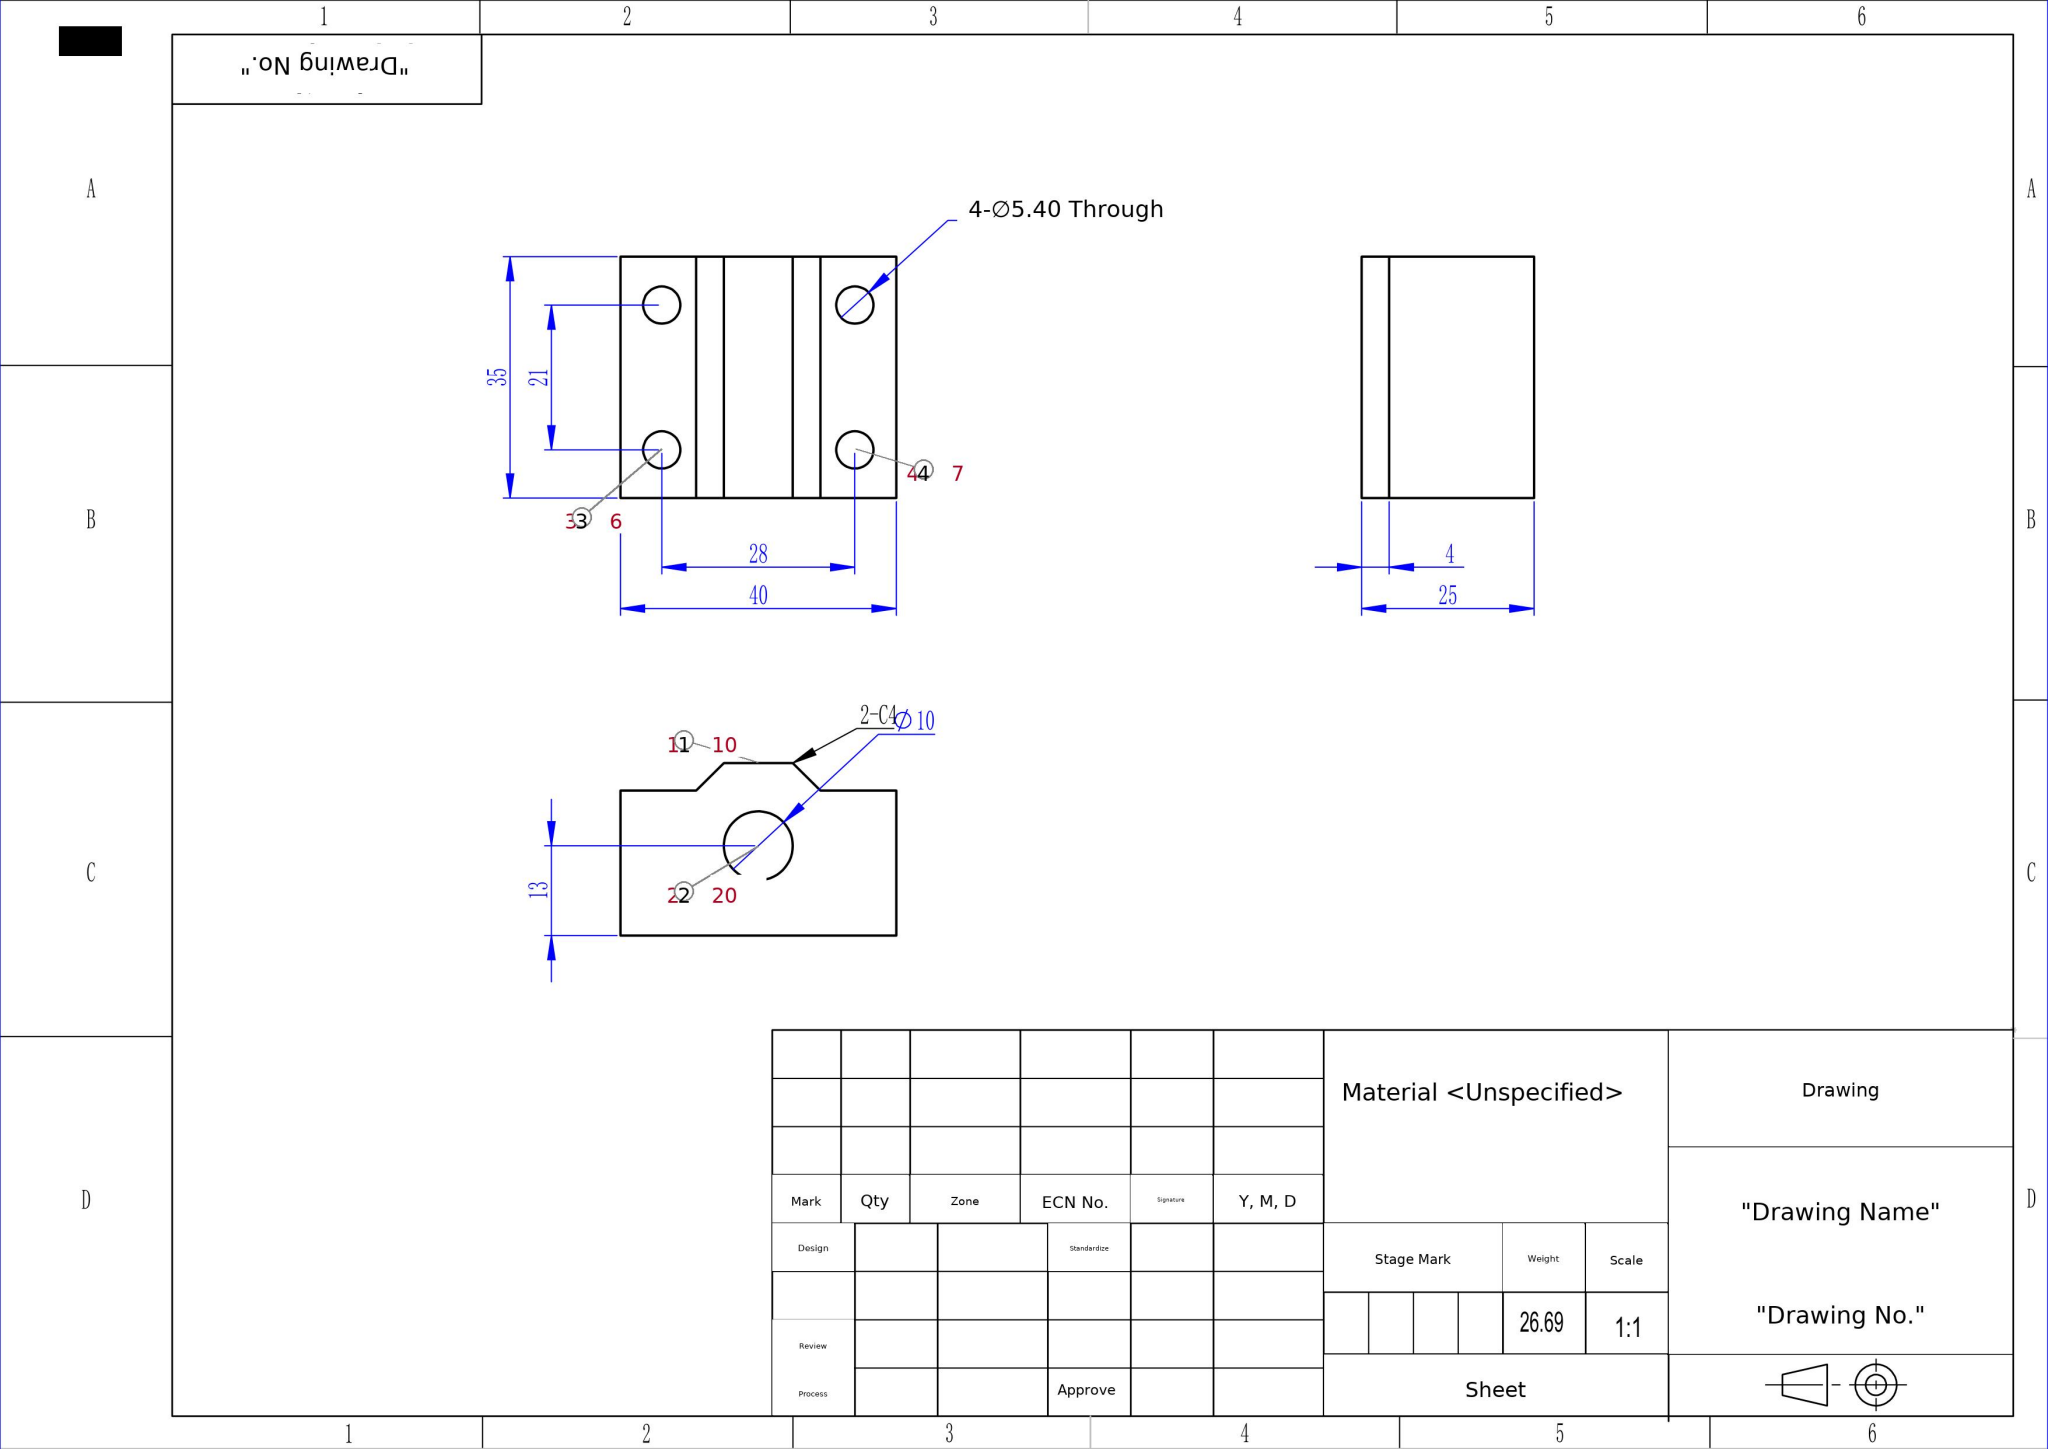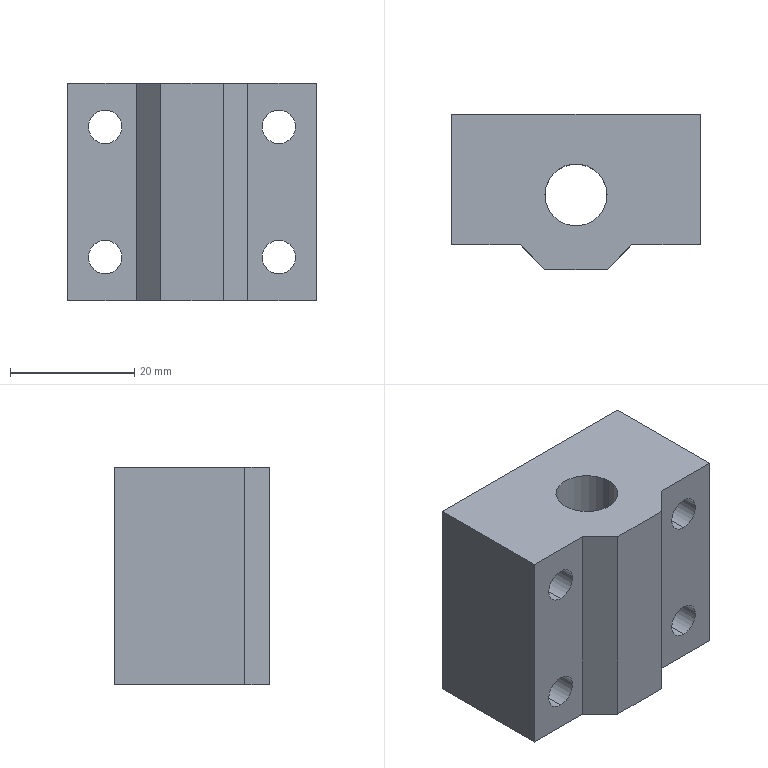Part | SolidWorks | mm | 1 solid | 20 faces | box 40 x 25 x 35 mm | volume 26687 mm3 | cylinder 10 | plane 10 | commonest cylinder face diameters 5.4 x8 10 x2
STEP:
#1=CARTESIAN_POINT('',(-14.,-8.,4.3));
#2=VERTEX_POINT('',#1);
#3=CARTESIAN_POINT('',(-14.,-8.,9.7));
#4=VERTEX_POINT('',#3);
#5=CARTESIAN_POINT('',(-14.,-8.,7.));
#6=DIRECTION('',(0.,1.,0.));
#7=DIRECTION('',(0.,0.,1.));
#8=AXIS2_PLACEMENT_3D('',#5,#6,#7);
#9=CIRCLE('',#8,2.7);
#10=EDGE_CURVE('',#2,#4,#9,.T.);
#11=ORIENTED_EDGE('',*,*,#10,.F.);
#12=CARTESIAN_POINT('',(-14.,13.,4.3));
#13=VERTEX_POINT('',#12);
#14=CARTESIAN_POINT('',(-14.,-12.,4.3));
#15=DIRECTION('',(0.,1.,0.));
#16=VECTOR('',#15,1000.);
#17=LINE('',#14,#16);
#18=EDGE_CURVE('',#2,#13,#17,.T.);
#19=ORIENTED_EDGE('',*,*,#18,.T.);
#20=CARTESIAN_POINT('',(-14.,13.,9.7));
#21=VERTEX_POINT('',#20);
#22=CARTESIAN_POINT('',(-14.,13.,7.));
#23=DIRECTION('',(0.,1.,0.));
#24=DIRECTION('',(0.,0.,1.));
#25=AXIS2_PLACEMENT_3D('',#22,#23,#24);
#26=CIRCLE('',#25,2.7);
#27=EDGE_CURVE('',#13,#21,#26,.T.);
#28=ORIENTED_EDGE('',*,*,#27,.T.);
#29=CARTESIAN_POINT('',(-14.,-12.,9.7));
#30=DIRECTION('',(0.,1.,0.));
#31=VECTOR('',#30,1000.);
#32=LINE('',#29,#31);
#33=EDGE_CURVE('',#4,#21,#32,.T.);
#34=ORIENTED_EDGE('',*,*,#33,.F.);
#35=EDGE_LOOP('',(#11,#19,#28,#34));
#36=FACE_OUTER_BOUND('',#35,.T.);
#37=CARTESIAN_POINT('',(-14.,-12.,7.));
#38=DIRECTION('',(0.,1.,0.));
#39=DIRECTION('',(0.,0.,1.));
#40=AXIS2_PLACEMENT_3D('',#37,#38,#39);
#41=CYLINDRICAL_SURFACE('',#40,2.7);
#42=ADVANCED_FACE('',(#36),#41,.F.);
#43=CARTESIAN_POINT('',(14.,-8.,4.3));
#44=VERTEX_POINT('',#43);
#45=CARTESIAN_POINT('',(14.,-8.,9.7));
#46=VERTEX_POINT('',#45);
#47=CARTESIAN_POINT('',(14.,-8.,7.));
#48=DIRECTION('',(0.,1.,0.));
#49=DIRECTION('',(0.,0.,1.));
#50=AXIS2_PLACEMENT_3D('',#47,#48,#49);
#51=CIRCLE('',#50,2.7);
#52=EDGE_CURVE('',#44,#46,#51,.T.);
#53=ORIENTED_EDGE('',*,*,#52,.F.);
#54=CARTESIAN_POINT('',(14.,13.,4.3));
#55=VERTEX_POINT('',#54);
#56=CARTESIAN_POINT('',(14.,-12.,4.3));
#57=DIRECTION('',(0.,1.,0.));
#58=VECTOR('',#57,1000.);
#59=LINE('',#56,#58);
#60=EDGE_CURVE('',#44,#55,#59,.T.);
#61=ORIENTED_EDGE('',*,*,#60,.T.);
#62=CARTESIAN_POINT('',(14.,13.,9.7));
#63=VERTEX_POINT('',#62);
#64=CARTESIAN_POINT('',(14.,13.,7.));
#65=DIRECTION('',(0.,1.,0.));
#66=DIRECTION('',(0.,0.,1.));
#67=AXIS2_PLACEMENT_3D('',#64,#65,#66);
#68=CIRCLE('',#67,2.7);
#69=EDGE_CURVE('',#55,#63,#68,.T.);
#70=ORIENTED_EDGE('',*,*,#69,.T.);
#71=CARTESIAN_POINT('',(14.,-12.,9.7));
#72=DIRECTION('',(0.,1.,0.));
#73=VECTOR('',#72,1000.);
#74=LINE('',#71,#73);
#75=EDGE_CURVE('',#46,#63,#74,.T.);
#76=ORIENTED_EDGE('',*,*,#75,.F.);
#77=EDGE_LOOP('',(#53,#61,#70,#76));
#78=FACE_OUTER_BOUND('',#77,.T.);
#79=CARTESIAN_POINT('',(14.,-12.,7.));
#80=DIRECTION('',(0.,1.,0.));
#81=DIRECTION('',(0.,0.,1.));
#82=AXIS2_PLACEMENT_3D('',#79,#80,#81);
#83=CYLINDRICAL_SURFACE('',#82,2.7);
#84=ADVANCED_FACE('',(#78),#83,.F.);
#85=CARTESIAN_POINT('',(14.,-8.,25.3));
#86=VERTEX_POINT('',#85);
#87=CARTESIAN_POINT('',(14.,-8.,30.7));
#88=VERTEX_POINT('',#87);
#89=CARTESIAN_POINT('',(14.,-8.,28.));
#90=DIRECTION('',(0.,1.,0.));
#91=DIRECTION('',(0.,0.,1.));
#92=AXIS2_PLACEMENT_3D('',#89,#90,#91);
#93=CIRCLE('',#92,2.7);
#94=EDGE_CURVE('',#86,#88,#93,.T.);
#95=ORIENTED_EDGE('',*,*,#94,.F.);
#96=CARTESIAN_POINT('',(14.,13.,25.3));
#97=VERTEX_POINT('',#96);
#98=CARTESIAN_POINT('',(14.,-12.,25.3));
#99=DIRECTION('',(0.,1.,0.));
#100=VECTOR('',#99,1000.);
#101=LINE('',#98,#100);
#102=EDGE_CURVE('',#86,#97,#101,.T.);
#103=ORIENTED_EDGE('',*,*,#102,.T.);
#104=CARTESIAN_POINT('',(14.,13.,30.7));
#105=VERTEX_POINT('',#104);
#106=CARTESIAN_POINT('',(14.,13.,28.));
#107=DIRECTION('',(0.,1.,0.));
#108=DIRECTION('',(0.,0.,1.));
#109=AXIS2_PLACEMENT_3D('',#106,#107,#108);
#110=CIRCLE('',#109,2.7);
#111=EDGE_CURVE('',#97,#105,#110,.T.);
#112=ORIENTED_EDGE('',*,*,#111,.T.);
#113=CARTESIAN_POINT('',(14.,-12.,30.7));
#114=DIRECTION('',(0.,1.,0.));
#115=VECTOR('',#114,1000.);
#116=LINE('',#113,#115);
#117=EDGE_CURVE('',#88,#105,#116,.T.);
#118=ORIENTED_EDGE('',*,*,#117,.F.);
#119=EDGE_LOOP('',(#95,#103,#112,#118));
#120=FACE_OUTER_BOUND('',#119,.T.);
#121=CARTESIAN_POINT('',(14.,-12.,28.));
#122=DIRECTION('',(0.,1.,0.));
#123=DIRECTION('',(0.,0.,1.));
#124=AXIS2_PLACEMENT_3D('',#121,#122,#123);
#125=CYLINDRICAL_SURFACE('',#124,2.7);
#126=ADVANCED_FACE('',(#120),#125,.F.);
#127=CARTESIAN_POINT('',(-14.,-8.,25.3));
#128=VERTEX_POINT('',#127);
#129=CARTESIAN_POINT('',(-14.,-8.,30.7));
#130=VERTEX_POINT('',#129);
#131=CARTESIAN_POINT('',(-14.,-8.,28.));
#132=DIRECTION('',(0.,1.,0.));
#133=DIRECTION('',(0.,0.,1.));
#134=AXIS2_PLACEMENT_3D('',#131,#132,#133);
#135=CIRCLE('',#134,2.7);
#136=EDGE_CURVE('',#128,#130,#135,.T.);
#137=ORIENTED_EDGE('',*,*,#136,.F.);
#138=CARTESIAN_POINT('',(-14.,13.,25.3));
#139=VERTEX_POINT('',#138);
#140=CARTESIAN_POINT('',(-14.,-12.,25.3));
#141=DIRECTION('',(0.,1.,0.));
#142=VECTOR('',#141,1000.);
#143=LINE('',#140,#142);
#144=EDGE_CURVE('',#128,#139,#143,.T.);
#145=ORIENTED_EDGE('',*,*,#144,.T.);
#146=CARTESIAN_POINT('',(-14.,13.,30.7));
#147=VERTEX_POINT('',#146);
#148=CARTESIAN_POINT('',(-14.,13.,28.));
#149=DIRECTION('',(0.,1.,0.));
#150=DIRECTION('',(0.,0.,1.));
#151=AXIS2_PLACEMENT_3D('',#148,#149,#150);
#152=CIRCLE('',#151,2.7);
#153=EDGE_CURVE('',#139,#147,#152,.T.);
#154=ORIENTED_EDGE('',*,*,#153,.T.);
#155=CARTESIAN_POINT('',(-14.,-12.,30.7));
#156=DIRECTION('',(0.,1.,0.));
#157=VECTOR('',#156,1000.);
#158=LINE('',#155,#157);
#159=EDGE_CURVE('',#130,#147,#158,.T.);
#160=ORIENTED_EDGE('',*,*,#159,.F.);
#161=EDGE_LOOP('',(#137,#145,#154,#160));
#162=FACE_OUTER_BOUND('',#161,.T.);
#163=CARTESIAN_POINT('',(-14.,-12.,28.));
#164=DIRECTION('',(0.,1.,0.));
#165=DIRECTION('',(0.,0.,1.));
#166=AXIS2_PLACEMENT_3D('',#163,#164,#165);
#167=CYLINDRICAL_SURFACE('',#166,2.7);
#168=ADVANCED_FACE('',(#162),#167,.F.);
#169=CARTESIAN_POINT('',(-5.,0.,35.));
#170=VERTEX_POINT('',#169);
#171=CARTESIAN_POINT('',(5.,0.,35.));
#172=VERTEX_POINT('',#171);
#173=CARTESIAN_POINT('',(0.,0.,35.));
#174=DIRECTION('',(0.,0.,1.));
#175=DIRECTION('',(1.,0.,0.));
#176=AXIS2_PLACEMENT_3D('',#173,#174,#175);
#177=CIRCLE('',#176,5.);
#178=EDGE_CURVE('',#170,#172,#177,.T.);
#179=ORIENTED_EDGE('',*,*,#178,.T.);
#180=CARTESIAN_POINT('',(5.,0.,0.));
#181=VERTEX_POINT('',#180);
#182=CARTESIAN_POINT('',(5.,0.,35.));
#183=DIRECTION('',(0.,0.,-1.));
#184=VECTOR('',#183,1000.);
#185=LINE('',#182,#184);
#186=EDGE_CURVE('',#172,#181,#185,.T.);
#187=ORIENTED_EDGE('',*,*,#186,.T.);
#188=CARTESIAN_POINT('',(-5.,0.,0.));
#189=VERTEX_POINT('',#188);
#190=CARTESIAN_POINT('',(0.,0.,0.));
#191=DIRECTION('',(0.,0.,1.));
#192=DIRECTION('',(1.,0.,0.));
#193=AXIS2_PLACEMENT_3D('',#190,#191,#192);
#194=CIRCLE('',#193,5.);
#195=EDGE_CURVE('',#189,#181,#194,.T.);
#196=ORIENTED_EDGE('',*,*,#195,.F.);
#197=CARTESIAN_POINT('',(-5.,0.,35.));
#198=DIRECTION('',(0.,0.,-1.));
#199=VECTOR('',#198,1000.);
#200=LINE('',#197,#199);
#201=EDGE_CURVE('',#170,#189,#200,.T.);
#202=ORIENTED_EDGE('',*,*,#201,.F.);
#203=EDGE_LOOP('',(#179,#187,#196,#202));
#204=FACE_OUTER_BOUND('',#203,.T.);
#205=CARTESIAN_POINT('',(0.,0.,35.));
#206=DIRECTION('',(0.,0.,-1.));
#207=DIRECTION('',(-1.,0.,0.));
#208=AXIS2_PLACEMENT_3D('',#205,#206,#207);
#209=CYLINDRICAL_SURFACE('',#208,5.);
#210=ADVANCED_FACE('',(#204),#209,.F.);
#211=CARTESIAN_POINT('',(-20.,13.,35.));
#212=VERTEX_POINT('',#211);
#213=CARTESIAN_POINT('',(-20.,-8.,35.));
#214=VERTEX_POINT('',#213);
#215=CARTESIAN_POINT('',(-20.,13.,35.));
#216=DIRECTION('',(0.,-1.,0.));
#217=VECTOR('',#216,1000.);
#218=LINE('',#215,#217);
#219=EDGE_CURVE('',#212,#214,#218,.T.);
#220=ORIENTED_EDGE('',*,*,#219,.T.);
#221=CARTESIAN_POINT('',(-9.,-8.,35.));
#222=VERTEX_POINT('',#221);
#223=CARTESIAN_POINT('',(-20.,-8.,35.));
#224=DIRECTION('',(1.,0.,0.));
#225=VECTOR('',#224,1000.);
#226=LINE('',#223,#225);
#227=EDGE_CURVE('',#214,#222,#226,.T.);
#228=ORIENTED_EDGE('',*,*,#227,.T.);
#229=CARTESIAN_POINT('',(-5.,-12.,35.));
#230=VERTEX_POINT('',#229);
#231=CARTESIAN_POINT('',(-5.,-12.,35.));
#232=DIRECTION('',(0.7071,-0.7071,0.));
#233=VECTOR('',#232,1000.);
#234=LINE('',#231,#233);
#235=EDGE_CURVE('',#222,#230,#234,.T.);
#236=ORIENTED_EDGE('',*,*,#235,.T.);
#237=CARTESIAN_POINT('',(5.,-12.,35.));
#238=VERTEX_POINT('',#237);
#239=CARTESIAN_POINT('',(-5.,-12.,35.));
#240=DIRECTION('',(1.,0.,0.));
#241=VECTOR('',#240,1000.);
#242=LINE('',#239,#241);
#243=EDGE_CURVE('',#230,#238,#242,.T.);
#244=ORIENTED_EDGE('',*,*,#243,.T.);
#245=CARTESIAN_POINT('',(9.,-8.,35.));
#246=VERTEX_POINT('',#245);
#247=CARTESIAN_POINT('',(9.,-8.,35.));
#248=DIRECTION('',(0.7071,0.7071,0.));
#249=VECTOR('',#248,1000.);
#250=LINE('',#247,#249);
#251=EDGE_CURVE('',#238,#246,#250,.T.);
#252=ORIENTED_EDGE('',*,*,#251,.T.);
#253=CARTESIAN_POINT('',(20.,-8.,35.));
#254=VERTEX_POINT('',#253);
#255=CARTESIAN_POINT('',(5.,-8.,35.));
#256=DIRECTION('',(1.,0.,0.));
#257=VECTOR('',#256,1000.);
#258=LINE('',#255,#257);
#259=EDGE_CURVE('',#246,#254,#258,.T.);
#260=ORIENTED_EDGE('',*,*,#259,.T.);
#261=CARTESIAN_POINT('',(20.,13.,35.));
#262=VERTEX_POINT('',#261);
#263=CARTESIAN_POINT('',(20.,13.,35.));
#264=DIRECTION('',(0.,1.,0.));
#265=VECTOR('',#264,1000.);
#266=LINE('',#263,#265);
#267=EDGE_CURVE('',#254,#262,#266,.T.);
#268=ORIENTED_EDGE('',*,*,#267,.T.);
#269=CARTESIAN_POINT('',(-20.,13.,35.));
#270=DIRECTION('',(-1.,0.,0.));
#271=VECTOR('',#270,1000.);
#272=LINE('',#269,#271);
#273=EDGE_CURVE('',#262,#212,#272,.T.);
#274=ORIENTED_EDGE('',*,*,#273,.T.);
#275=EDGE_LOOP('',(#220,#228,#236,#244,#252,#260,#268,#274));
#276=FACE_OUTER_BOUND('',#275,.T.);
#277=ORIENTED_EDGE('',*,*,#178,.F.);
#278=CARTESIAN_POINT('',(0.,0.,35.));
#279=DIRECTION('',(0.,0.,1.));
#280=DIRECTION('',(1.,0.,0.));
#281=AXIS2_PLACEMENT_3D('',#278,#279,#280);
#282=CIRCLE('',#281,5.);
#283=EDGE_CURVE('',#172,#170,#282,.T.);
#284=ORIENTED_EDGE('',*,*,#283,.F.);
#285=EDGE_LOOP('',(#277,#284));
#286=FACE_BOUND('',#285,.T.);
#287=CARTESIAN_POINT('',(0.,0.,35.));
#288=DIRECTION('',(0.,0.,1.));
#289=DIRECTION('',(1.,0.,0.));
#290=AXIS2_PLACEMENT_3D('',#287,#288,#289);
#291=PLANE('',#290);
#292=ADVANCED_FACE('',(#276,#286),#291,.T.);
#293=CARTESIAN_POINT('',(-20.,13.,0.));
#294=VERTEX_POINT('',#293);
#295=CARTESIAN_POINT('',(-20.,-8.,0.));
#296=VERTEX_POINT('',#295);
#297=CARTESIAN_POINT('',(-20.,13.,0.));
#298=DIRECTION('',(0.,-1.,0.));
#299=VECTOR('',#298,1000.);
#300=LINE('',#297,#299);
#301=EDGE_CURVE('',#294,#296,#300,.T.);
#302=ORIENTED_EDGE('',*,*,#301,.F.);
#303=CARTESIAN_POINT('',(20.,13.,0.));
#304=VERTEX_POINT('',#303);
#305=CARTESIAN_POINT('',(-20.,13.,0.));
#306=DIRECTION('',(-1.,0.,0.));
#307=VECTOR('',#306,1000.);
#308=LINE('',#305,#307);
#309=EDGE_CURVE('',#304,#294,#308,.T.);
#310=ORIENTED_EDGE('',*,*,#309,.F.);
#311=CARTESIAN_POINT('',(20.,-8.,0.));
#312=VERTEX_POINT('',#311);
#313=CARTESIAN_POINT('',(20.,13.,0.));
#314=DIRECTION('',(0.,1.,0.));
#315=VECTOR('',#314,1000.);
#316=LINE('',#313,#315);
#317=EDGE_CURVE('',#312,#304,#316,.T.);
#318=ORIENTED_EDGE('',*,*,#317,.F.);
#319=CARTESIAN_POINT('',(9.,-8.,0.));
#320=VERTEX_POINT('',#319);
#321=CARTESIAN_POINT('',(5.,-8.,0.));
#322=DIRECTION('',(1.,0.,0.));
#323=VECTOR('',#322,1000.);
#324=LINE('',#321,#323);
#325=EDGE_CURVE('',#320,#312,#324,.T.);
#326=ORIENTED_EDGE('',*,*,#325,.F.);
#327=CARTESIAN_POINT('',(5.,-12.,0.));
#328=VERTEX_POINT('',#327);
#329=CARTESIAN_POINT('',(8.5,-8.5,0.));
#330=DIRECTION('',(-0.7071,-0.7071,0.));
#331=VECTOR('',#330,1000.);
#332=LINE('',#329,#331);
#333=EDGE_CURVE('',#320,#328,#332,.T.);
#334=ORIENTED_EDGE('',*,*,#333,.T.);
#335=CARTESIAN_POINT('',(-5.,-12.,0.));
#336=VERTEX_POINT('',#335);
#337=CARTESIAN_POINT('',(-5.,-12.,0.));
#338=DIRECTION('',(1.,0.,0.));
#339=VECTOR('',#338,1000.);
#340=LINE('',#337,#339);
#341=EDGE_CURVE('',#336,#328,#340,.T.);
#342=ORIENTED_EDGE('',*,*,#341,.F.);
#343=CARTESIAN_POINT('',(-9.,-8.,0.));
#344=VERTEX_POINT('',#343);
#345=CARTESIAN_POINT('',(-8.5,-8.5,0.));
#346=DIRECTION('',(-0.7071,0.7071,0.));
#347=VECTOR('',#346,1000.);
#348=LINE('',#345,#347);
#349=EDGE_CURVE('',#336,#344,#348,.T.);
#350=ORIENTED_EDGE('',*,*,#349,.T.);
#351=CARTESIAN_POINT('',(-20.,-8.,0.));
#352=DIRECTION('',(1.,0.,0.));
#353=VECTOR('',#352,1000.);
#354=LINE('',#351,#353);
#355=EDGE_CURVE('',#296,#344,#354,.T.);
#356=ORIENTED_EDGE('',*,*,#355,.F.);
#357=EDGE_LOOP('',(#302,#310,#318,#326,#334,#342,#350,#356));
#358=FACE_OUTER_BOUND('',#357,.T.);
#359=ORIENTED_EDGE('',*,*,#195,.T.);
#360=CARTESIAN_POINT('',(0.,0.,0.));
#361=DIRECTION('',(0.,0.,1.));
#362=DIRECTION('',(1.,0.,0.));
#363=AXIS2_PLACEMENT_3D('',#360,#361,#362);
#364=CIRCLE('',#363,5.);
#365=EDGE_CURVE('',#181,#189,#364,.T.);
#366=ORIENTED_EDGE('',*,*,#365,.T.);
#367=EDGE_LOOP('',(#359,#366));
#368=FACE_BOUND('',#367,.T.);
#369=CARTESIAN_POINT('',(0.,0.,0.));
#370=DIRECTION('',(0.,0.,1.));
#371=DIRECTION('',(1.,0.,0.));
#372=AXIS2_PLACEMENT_3D('',#369,#370,#371);
#373=PLANE('',#372);
#374=ADVANCED_FACE('',(#358,#368),#373,.F.);
#375=ORIENTED_EDGE('',*,*,#301,.T.);
#376=CARTESIAN_POINT('',(-20.,-8.,35.));
#377=DIRECTION('',(0.,0.,-1.));
#378=VECTOR('',#377,1000.);
#379=LINE('',#376,#378);
#380=EDGE_CURVE('',#214,#296,#379,.T.);
#381=ORIENTED_EDGE('',*,*,#380,.F.);
#382=ORIENTED_EDGE('',*,*,#219,.F.);
#383=CARTESIAN_POINT('',(-20.,13.,35.));
#384=DIRECTION('',(0.,0.,-1.));
#385=VECTOR('',#384,1000.);
#386=LINE('',#383,#385);
#387=EDGE_CURVE('',#212,#294,#386,.T.);
#388=ORIENTED_EDGE('',*,*,#387,.T.);
#389=EDGE_LOOP('',(#375,#381,#382,#388));
#390=FACE_OUTER_BOUND('',#389,.T.);
#391=CARTESIAN_POINT('',(-20.,13.,35.));
#392=DIRECTION('',(1.,0.,0.));
#393=DIRECTION('',(-0.,1.,0.));
#394=AXIS2_PLACEMENT_3D('',#391,#392,#393);
#395=PLANE('',#394);
#396=ADVANCED_FACE('',(#390),#395,.F.);
#397=CARTESIAN_POINT('',(-14.,-8.,7.));
#398=DIRECTION('',(0.,1.,0.));
#399=DIRECTION('',(0.,0.,1.));
#400=AXIS2_PLACEMENT_3D('',#397,#398,#399);
#401=CIRCLE('',#400,2.7);
#402=EDGE_CURVE('',#4,#2,#401,.T.);
#403=ORIENTED_EDGE('',*,*,#402,.T.);
#404=ORIENTED_EDGE('',*,*,#10,.T.);
#405=EDGE_LOOP('',(#403,#404));
#406=FACE_BOUND('',#405,.T.);
#407=CARTESIAN_POINT('',(-14.,-8.,28.));
#408=DIRECTION('',(0.,1.,0.));
#409=DIRECTION('',(0.,0.,1.));
#410=AXIS2_PLACEMENT_3D('',#407,#408,#409);
#411=CIRCLE('',#410,2.7);
#412=EDGE_CURVE('',#130,#128,#411,.T.);
#413=ORIENTED_EDGE('',*,*,#412,.T.);
#414=ORIENTED_EDGE('',*,*,#136,.T.);
#415=EDGE_LOOP('',(#413,#414));
#416=FACE_BOUND('',#415,.T.);
#417=ORIENTED_EDGE('',*,*,#355,.T.);
#418=CARTESIAN_POINT('',(-9.,-8.,35.));
#419=DIRECTION('',(0.,0.,1.));
#420=VECTOR('',#419,1000.);
#421=LINE('',#418,#420);
#422=EDGE_CURVE('',#344,#222,#421,.T.);
#423=ORIENTED_EDGE('',*,*,#422,.T.);
#424=ORIENTED_EDGE('',*,*,#227,.F.);
#425=ORIENTED_EDGE('',*,*,#380,.T.);
#426=EDGE_LOOP('',(#417,#423,#424,#425));
#427=FACE_OUTER_BOUND('',#426,.T.);
#428=CARTESIAN_POINT('',(-20.,-8.,35.));
#429=DIRECTION('',(0.,1.,0.));
#430=DIRECTION('',(0.,0.,1.));
#431=AXIS2_PLACEMENT_3D('',#428,#429,#430);
#432=PLANE('',#431);
#433=ADVANCED_FACE('',(#406,#416,#427),#432,.F.);
#434=ORIENTED_EDGE('',*,*,#341,.T.);
#435=CARTESIAN_POINT('',(5.,-12.,35.));
#436=DIRECTION('',(0.,0.,-1.));
#437=VECTOR('',#436,1000.);
#438=LINE('',#435,#437);
#439=EDGE_CURVE('',#238,#328,#438,.T.);
#440=ORIENTED_EDGE('',*,*,#439,.F.);
#441=ORIENTED_EDGE('',*,*,#243,.F.);
#442=CARTESIAN_POINT('',(-5.,-12.,35.));
#443=DIRECTION('',(0.,0.,-1.));
#444=VECTOR('',#443,1000.);
#445=LINE('',#442,#444);
#446=EDGE_CURVE('',#230,#336,#445,.T.);
#447=ORIENTED_EDGE('',*,*,#446,.T.);
#448=EDGE_LOOP('',(#434,#440,#441,#447));
#449=FACE_OUTER_BOUND('',#448,.T.);
#450=CARTESIAN_POINT('',(-5.,-12.,35.));
#451=DIRECTION('',(0.,1.,0.));
#452=DIRECTION('',(0.,0.,1.));
#453=AXIS2_PLACEMENT_3D('',#450,#451,#452);
#454=PLANE('',#453);
#455=ADVANCED_FACE('',(#449),#454,.F.);
#456=CARTESIAN_POINT('',(14.,-8.,7.));
#457=DIRECTION('',(0.,1.,0.));
#458=DIRECTION('',(0.,0.,1.));
#459=AXIS2_PLACEMENT_3D('',#456,#457,#458);
#460=CIRCLE('',#459,2.7);
#461=EDGE_CURVE('',#46,#44,#460,.T.);
#462=ORIENTED_EDGE('',*,*,#461,.T.);
#463=ORIENTED_EDGE('',*,*,#52,.T.);
#464=EDGE_LOOP('',(#462,#463));
#465=FACE_BOUND('',#464,.T.);
#466=CARTESIAN_POINT('',(14.,-8.,28.));
#467=DIRECTION('',(0.,1.,0.));
#468=DIRECTION('',(0.,0.,1.));
#469=AXIS2_PLACEMENT_3D('',#466,#467,#468);
#470=CIRCLE('',#469,2.7);
#471=EDGE_CURVE('',#88,#86,#470,.T.);
#472=ORIENTED_EDGE('',*,*,#471,.T.);
#473=ORIENTED_EDGE('',*,*,#94,.T.);
#474=EDGE_LOOP('',(#472,#473));
#475=FACE_BOUND('',#474,.T.);
#476=ORIENTED_EDGE('',*,*,#259,.F.);
#477=CARTESIAN_POINT('',(9.,-8.,0.));
#478=DIRECTION('',(0.,0.,-1.));
#479=VECTOR('',#478,1000.);
#480=LINE('',#477,#479);
#481=EDGE_CURVE('',#246,#320,#480,.T.);
#482=ORIENTED_EDGE('',*,*,#481,.T.);
#483=ORIENTED_EDGE('',*,*,#325,.T.);
#484=CARTESIAN_POINT('',(20.,-8.,35.));
#485=DIRECTION('',(0.,0.,-1.));
#486=VECTOR('',#485,1000.);
#487=LINE('',#484,#486);
#488=EDGE_CURVE('',#254,#312,#487,.T.);
#489=ORIENTED_EDGE('',*,*,#488,.F.);
#490=EDGE_LOOP('',(#476,#482,#483,#489));
#491=FACE_OUTER_BOUND('',#490,.T.);
#492=CARTESIAN_POINT('',(5.,-8.,35.));
#493=DIRECTION('',(0.,1.,0.));
#494=DIRECTION('',(0.,0.,1.));
#495=AXIS2_PLACEMENT_3D('',#492,#493,#494);
#496=PLANE('',#495);
#497=ADVANCED_FACE('',(#465,#475,#491),#496,.F.);
#498=ORIENTED_EDGE('',*,*,#317,.T.);
#499=CARTESIAN_POINT('',(20.,13.,35.));
#500=DIRECTION('',(0.,0.,-1.));
#501=VECTOR('',#500,1000.);
#502=LINE('',#499,#501);
#503=EDGE_CURVE('',#262,#304,#502,.T.);
#504=ORIENTED_EDGE('',*,*,#503,.F.);
#505=ORIENTED_EDGE('',*,*,#267,.F.);
#506=ORIENTED_EDGE('',*,*,#488,.T.);
#507=EDGE_LOOP('',(#498,#504,#505,#506));
#508=FACE_OUTER_BOUND('',#507,.T.);
#509=CARTESIAN_POINT('',(20.,13.,35.));
#510=DIRECTION('',(-1.,0.,0.));
#511=DIRECTION('',(-0.,-1.,0.));
#512=AXIS2_PLACEMENT_3D('',#509,#510,#511);
#513=PLANE('',#512);
#514=ADVANCED_FACE('',(#508),#513,.F.);
#515=CARTESIAN_POINT('',(-14.,13.,7.));
#516=DIRECTION('',(0.,1.,0.));
#517=DIRECTION('',(0.,0.,1.));
#518=AXIS2_PLACEMENT_3D('',#515,#516,#517);
#519=CIRCLE('',#518,2.7);
#520=EDGE_CURVE('',#21,#13,#519,.T.);
#521=ORIENTED_EDGE('',*,*,#520,.F.);
#522=ORIENTED_EDGE('',*,*,#27,.F.);
#523=EDGE_LOOP('',(#521,#522));
#524=FACE_BOUND('',#523,.T.);
#525=CARTESIAN_POINT('',(14.,13.,7.));
#526=DIRECTION('',(0.,1.,0.));
#527=DIRECTION('',(0.,0.,1.));
#528=AXIS2_PLACEMENT_3D('',#525,#526,#527);
#529=CIRCLE('',#528,2.7);
#530=EDGE_CURVE('',#63,#55,#529,.T.);
#531=ORIENTED_EDGE('',*,*,#530,.F.);
#532=ORIENTED_EDGE('',*,*,#69,.F.);
#533=EDGE_LOOP('',(#531,#532));
#534=FACE_BOUND('',#533,.T.);
#535=CARTESIAN_POINT('',(14.,13.,28.));
#536=DIRECTION('',(0.,1.,0.));
#537=DIRECTION('',(0.,0.,1.));
#538=AXIS2_PLACEMENT_3D('',#535,#536,#537);
#539=CIRCLE('',#538,2.7);
#540=EDGE_CURVE('',#105,#97,#539,.T.);
#541=ORIENTED_EDGE('',*,*,#540,.F.);
#542=ORIENTED_EDGE('',*,*,#111,.F.);
#543=EDGE_LOOP('',(#541,#542));
#544=FACE_BOUND('',#543,.T.);
#545=CARTESIAN_POINT('',(-14.,13.,28.));
#546=DIRECTION('',(0.,1.,0.));
#547=DIRECTION('',(0.,0.,1.));
#548=AXIS2_PLACEMENT_3D('',#545,#546,#547);
#549=CIRCLE('',#548,2.7);
#550=EDGE_CURVE('',#147,#139,#549,.T.);
#551=ORIENTED_EDGE('',*,*,#550,.F.);
#552=ORIENTED_EDGE('',*,*,#153,.F.);
#553=EDGE_LOOP('',(#551,#552));
#554=FACE_BOUND('',#553,.T.);
#555=ORIENTED_EDGE('',*,*,#309,.T.);
#556=ORIENTED_EDGE('',*,*,#387,.F.);
#557=ORIENTED_EDGE('',*,*,#273,.F.);
#558=ORIENTED_EDGE('',*,*,#503,.T.);
#559=EDGE_LOOP('',(#555,#556,#557,#558));
#560=FACE_OUTER_BOUND('',#559,.T.);
#561=CARTESIAN_POINT('',(-20.,13.,35.));
#562=DIRECTION('',(0.,-1.,0.));
#563=DIRECTION('',(0.,0.,-1.));
#564=AXIS2_PLACEMENT_3D('',#561,#562,#563);
#565=PLANE('',#564);
#566=ADVANCED_FACE('',(#524,#534,#544,#554,#560),#565,.F.);
#567=ORIENTED_EDGE('',*,*,#186,.F.);
#568=ORIENTED_EDGE('',*,*,#283,.T.);
#569=ORIENTED_EDGE('',*,*,#201,.T.);
#570=ORIENTED_EDGE('',*,*,#365,.F.);
#571=EDGE_LOOP('',(#567,#568,#569,#570));
#572=FACE_OUTER_BOUND('',#571,.T.);
#573=CARTESIAN_POINT('',(0.,0.,35.));
#574=DIRECTION('',(0.,0.,-1.));
#575=DIRECTION('',(-1.,0.,0.));
#576=AXIS2_PLACEMENT_3D('',#573,#574,#575);
#577=CYLINDRICAL_SURFACE('',#576,5.);
#578=ADVANCED_FACE('',(#572),#577,.F.);
#579=ORIENTED_EDGE('',*,*,#251,.F.);
#580=ORIENTED_EDGE('',*,*,#439,.T.);
#581=ORIENTED_EDGE('',*,*,#333,.F.);
#582=ORIENTED_EDGE('',*,*,#481,.F.);
#583=EDGE_LOOP('',(#579,#580,#581,#582));
#584=FACE_OUTER_BOUND('',#583,.T.);
#585=CARTESIAN_POINT('',(9.,-8.,35.));
#586=DIRECTION('',(0.7071,-0.7071,0.));
#587=DIRECTION('',(0.,0.,1.));
#588=AXIS2_PLACEMENT_3D('',#585,#586,#587);
#589=PLANE('',#588);
#590=ADVANCED_FACE('',(#584),#589,.T.);
#591=ORIENTED_EDGE('',*,*,#235,.F.);
#592=ORIENTED_EDGE('',*,*,#422,.F.);
#593=ORIENTED_EDGE('',*,*,#349,.F.);
#594=ORIENTED_EDGE('',*,*,#446,.F.);
#595=EDGE_LOOP('',(#591,#592,#593,#594));
#596=FACE_OUTER_BOUND('',#595,.T.);
#597=CARTESIAN_POINT('',(-5.,-12.,35.));
#598=DIRECTION('',(-0.7071,-0.7071,0.));
#599=DIRECTION('',(0.,0.,1.));
#600=AXIS2_PLACEMENT_3D('',#597,#598,#599);
#601=PLANE('',#600);
#602=ADVANCED_FACE('',(#596),#601,.T.);
#603=ORIENTED_EDGE('',*,*,#144,.F.);
#604=ORIENTED_EDGE('',*,*,#412,.F.);
#605=ORIENTED_EDGE('',*,*,#159,.T.);
#606=ORIENTED_EDGE('',*,*,#550,.T.);
#607=EDGE_LOOP('',(#603,#604,#605,#606));
#608=FACE_OUTER_BOUND('',#607,.T.);
#609=CARTESIAN_POINT('',(-14.,-12.,28.));
#610=DIRECTION('',(0.,1.,0.));
#611=DIRECTION('',(0.,0.,1.));
#612=AXIS2_PLACEMENT_3D('',#609,#610,#611);
#613=CYLINDRICAL_SURFACE('',#612,2.7);
#614=ADVANCED_FACE('',(#608),#613,.F.);
#615=ORIENTED_EDGE('',*,*,#102,.F.);
#616=ORIENTED_EDGE('',*,*,#471,.F.);
#617=ORIENTED_EDGE('',*,*,#117,.T.);
#618=ORIENTED_EDGE('',*,*,#540,.T.);
#619=EDGE_LOOP('',(#615,#616,#617,#618));
#620=FACE_OUTER_BOUND('',#619,.T.);
#621=CARTESIAN_POINT('',(14.,-12.,28.));
#622=DIRECTION('',(0.,1.,0.));
#623=DIRECTION('',(0.,0.,1.));
#624=AXIS2_PLACEMENT_3D('',#621,#622,#623);
#625=CYLINDRICAL_SURFACE('',#624,2.7);
#626=ADVANCED_FACE('',(#620),#625,.F.);
#627=ORIENTED_EDGE('',*,*,#60,.F.);
#628=ORIENTED_EDGE('',*,*,#461,.F.);
#629=ORIENTED_EDGE('',*,*,#75,.T.);
#630=ORIENTED_EDGE('',*,*,#530,.T.);
#631=EDGE_LOOP('',(#627,#628,#629,#630));
#632=FACE_OUTER_BOUND('',#631,.T.);
#633=CARTESIAN_POINT('',(14.,-12.,7.));
#634=DIRECTION('',(0.,1.,0.));
#635=DIRECTION('',(0.,0.,1.));
#636=AXIS2_PLACEMENT_3D('',#633,#634,#635);
#637=CYLINDRICAL_SURFACE('',#636,2.7);
#638=ADVANCED_FACE('',(#632),#637,.F.);
#639=ORIENTED_EDGE('',*,*,#18,.F.);
#640=ORIENTED_EDGE('',*,*,#402,.F.);
#641=ORIENTED_EDGE('',*,*,#33,.T.);
#642=ORIENTED_EDGE('',*,*,#520,.T.);
#643=EDGE_LOOP('',(#639,#640,#641,#642));
#644=FACE_OUTER_BOUND('',#643,.T.);
#645=CARTESIAN_POINT('',(-14.,-12.,7.));
#646=DIRECTION('',(0.,1.,0.));
#647=DIRECTION('',(0.,0.,1.));
#648=AXIS2_PLACEMENT_3D('',#645,#646,#647);
#649=CYLINDRICAL_SURFACE('',#648,2.7);
#650=ADVANCED_FACE('',(#644),#649,.F.);
#651=CLOSED_SHELL('',(#42,#84,#126,#168,#210,#292,#374,#396,#433,#455,#497,#514,#566,#578,#590,#602,#614,#626,#638,#650));
#652=MANIFOLD_SOLID_BREP('',#651);
#653=CARTESIAN_POINT('',(0.,0.,0.));
#654=DIRECTION('',(0.,0.,1.));
#655=DIRECTION('',(1.,0.,0.));
#656=AXIS2_PLACEMENT_3D('',#653,#654,#655);
#657=(LENGTH_UNIT()NAMED_UNIT(*)SI_UNIT(.MILLI.,.METRE.));
#658=UNCERTAINTY_MEASURE_WITH_UNIT(LENGTH_MEASURE(0.00001),#657,'','');
#659=(NAMED_UNIT(*)PLANE_ANGLE_UNIT()SI_UNIT($,.RADIAN.));
#660=(NAMED_UNIT(*)SI_UNIT($,.STERADIAN.)SOLID_ANGLE_UNIT());
#661=(GEOMETRIC_REPRESENTATION_CONTEXT(3)GLOBAL_UNCERTAINTY_ASSIGNED_CONTEXT((#658))GLOBAL_UNIT_ASSIGNED_CONTEXT((#657,#659,#660))REPRESENTATION_CONTEXT('',''));
#662=ADVANCED_BREP_SHAPE_REPRESENTATION('',(#652,#656),#661);